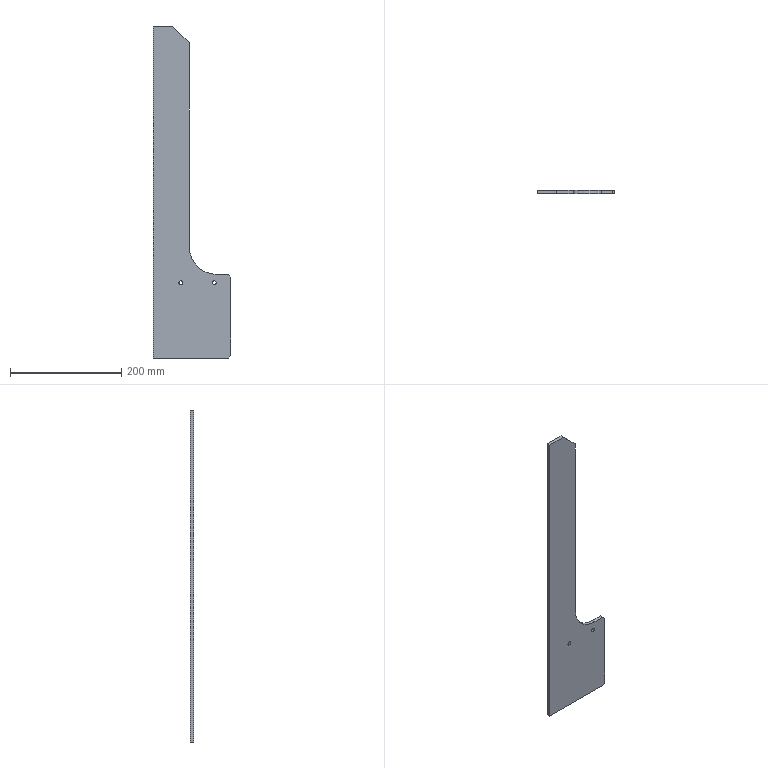Component | SolidWorks | THK-A1012BottomRibPlateRight-3 | 1 solid | 16 faces | box 140 x 6 x 596 mm | volume 299873 mm3 | plane 11 | cylinder 5 | commonest cylinder face diameters 6.8 x4 100 x1 | material Q235A
build123d program:
from build123d import *

# Parameters (mm, degrees)
BOSS_EXTRUDE1_DEPTH = 3
M8_TAPPED_HOLE1_D   = 6.8
CHAMFER2_SIZE       = 5
CHAMFER1_SIZE       = 30


with BuildPart() as part:
    # Sketch1 → Boss-Extrude1 (new, symmetric)
    with BuildSketch(Plane(origin=(0, 0, 0), x_dir=(1, 0, 0), z_dir=(0, 1, 0))):
        with BuildLine():
            Line((0, 0), (0, -596))
            Line((0, -596), (-65, -596))
            Line((-65, -596), (-65, -200))
            ThreePointArc((-65, -200), (-79.645, -164.645), (-115, -150))
            Line((-115, -150), (-140, -150))
            Line((-140, -150), (-140, 0))
            Line((-140, 0), (0, 0))
        make_face()
    extrude(amount=BOSS_EXTRUDE1_DEPTH, both=True)

    # M8 Tapped Hole1 (through all)
    with Locations(Plane(origin=(0, 3, 0), x_dir=(1, 0, 0), z_dir=(0, 1, 0))):
        with Locations((-110, -135), (-50, -135)):
            Hole(M8_TAPPED_HOLE1_D / 2)

    # Chamfer2
    chamfer2_edges = [part.edges().sort_by_distance(p)[0] for p in [
        (-140, 0, 150),
        (-140, 0, 0),
    ]]
    chamfer(chamfer2_edges, length=CHAMFER2_SIZE)

    # Chamfer1
    chamfer1_edges = [part.edges().sort_by_distance(p)[0] for p in [
        (-65, 0, 596),
    ]]
    chamfer(chamfer1_edges, length=CHAMFER1_SIZE)


solid = part.part

# Placed as in the assembly
solid = solid.moved(Location((73, -158, -371), (0, 0, 180)))
STEP:
#1=CARTESIAN_POINT('',(7.205,-6.102,-9.425));
#2=VERTEX_POINT('',#1);
#3=CARTESIAN_POINT('',(7.205,-6.102,-9.157));
#4=VERTEX_POINT('',#3);
#5=CARTESIAN_POINT('',(7.205,-6.102,-9.291));
#6=DIRECTION('',(0.,-1.,0.));
#7=DIRECTION('',(0.,0.,1.));
#8=AXIS2_PLACEMENT_3D('',#5,#6,#7);
#9=CIRCLE('',#8,0.1339);
#10=EDGE_CURVE('',#2,#4,#9,.T.);
#11=ORIENTED_EDGE('',*,*,#10,.F.);
#12=CARTESIAN_POINT('',(7.205,-6.339,-9.425));
#13=VERTEX_POINT('',#12);
#14=CARTESIAN_POINT('',(7.205,-6.339,-9.425));
#15=DIRECTION('',(0.,-1.,0.));
#16=VECTOR('',#15,39.37);
#17=LINE('',#14,#16);
#18=EDGE_CURVE('',#2,#13,#17,.T.);
#19=ORIENTED_EDGE('',*,*,#18,.T.);
#20=CARTESIAN_POINT('',(7.205,-6.339,-9.157));
#21=VERTEX_POINT('',#20);
#22=CARTESIAN_POINT('',(7.205,-6.339,-9.291));
#23=DIRECTION('',(0.,-1.,0.));
#24=DIRECTION('',(0.,0.,1.));
#25=AXIS2_PLACEMENT_3D('',#22,#23,#24);
#26=CIRCLE('',#25,0.1339);
#27=EDGE_CURVE('',#13,#21,#26,.T.);
#28=ORIENTED_EDGE('',*,*,#27,.T.);
#29=CARTESIAN_POINT('',(7.205,-6.339,-9.157));
#30=DIRECTION('',(0.,-1.,0.));
#31=VECTOR('',#30,39.37);
#32=LINE('',#29,#31);
#33=EDGE_CURVE('',#4,#21,#32,.T.);
#34=ORIENTED_EDGE('',*,*,#33,.F.);
#35=EDGE_LOOP('',(#11,#19,#28,#34));
#36=FACE_OUTER_BOUND('',#35,.T.);
#37=CARTESIAN_POINT('',(7.205,-6.339,-9.291));
#38=DIRECTION('',(0.,-1.,0.));
#39=DIRECTION('',(0.,0.,1.));
#40=AXIS2_PLACEMENT_3D('',#37,#38,#39);
#41=CYLINDRICAL_SURFACE('',#40,0.1339);
#42=ADVANCED_FACE('',(#36),#41,.F.);
#43=CARTESIAN_POINT('',(4.843,-6.102,-9.425));
#44=VERTEX_POINT('',#43);
#45=CARTESIAN_POINT('',(4.843,-6.102,-9.157));
#46=VERTEX_POINT('',#45);
#47=CARTESIAN_POINT('',(4.843,-6.102,-9.291));
#48=DIRECTION('',(0.,-1.,0.));
#49=DIRECTION('',(0.,0.,1.));
#50=AXIS2_PLACEMENT_3D('',#47,#48,#49);
#51=CIRCLE('',#50,0.1339);
#52=EDGE_CURVE('',#44,#46,#51,.T.);
#53=ORIENTED_EDGE('',*,*,#52,.F.);
#54=CARTESIAN_POINT('',(4.843,-6.339,-9.425));
#55=VERTEX_POINT('',#54);
#56=CARTESIAN_POINT('',(4.843,-6.339,-9.425));
#57=DIRECTION('',(0.,-1.,0.));
#58=VECTOR('',#57,39.37);
#59=LINE('',#56,#58);
#60=EDGE_CURVE('',#44,#55,#59,.T.);
#61=ORIENTED_EDGE('',*,*,#60,.T.);
#62=CARTESIAN_POINT('',(4.843,-6.339,-9.157));
#63=VERTEX_POINT('',#62);
#64=CARTESIAN_POINT('',(4.843,-6.339,-9.291));
#65=DIRECTION('',(0.,-1.,0.));
#66=DIRECTION('',(0.,0.,1.));
#67=AXIS2_PLACEMENT_3D('',#64,#65,#66);
#68=CIRCLE('',#67,0.1339);
#69=EDGE_CURVE('',#55,#63,#68,.T.);
#70=ORIENTED_EDGE('',*,*,#69,.T.);
#71=CARTESIAN_POINT('',(4.843,-6.339,-9.157));
#72=DIRECTION('',(0.,-1.,0.));
#73=VECTOR('',#72,39.37);
#74=LINE('',#71,#73);
#75=EDGE_CURVE('',#46,#63,#74,.T.);
#76=ORIENTED_EDGE('',*,*,#75,.F.);
#77=EDGE_LOOP('',(#53,#61,#70,#76));
#78=FACE_OUTER_BOUND('',#77,.T.);
#79=CARTESIAN_POINT('',(4.843,-6.339,-9.291));
#80=DIRECTION('',(0.,-1.,0.));
#81=DIRECTION('',(0.,0.,1.));
#82=AXIS2_PLACEMENT_3D('',#79,#80,#81);
#83=CYLINDRICAL_SURFACE('',#82,0.1339);
#84=ADVANCED_FACE('',(#78),#83,.F.);
#85=CARTESIAN_POINT('',(2.874,-6.102,-14.606));
#86=VERTEX_POINT('',#85);
#87=CARTESIAN_POINT('',(8.189,-6.102,-14.606));
#88=VERTEX_POINT('',#87);
#89=CARTESIAN_POINT('',(2.874,-6.102,-14.606));
#90=DIRECTION('',(1.,0.,-0.));
#91=VECTOR('',#90,39.37);
#92=LINE('',#89,#91);
#93=EDGE_CURVE('',#86,#88,#92,.T.);
#94=ORIENTED_EDGE('',*,*,#93,.T.);
#95=CARTESIAN_POINT('',(8.189,-6.339,-14.606));
#96=VERTEX_POINT('',#95);
#97=CARTESIAN_POINT('',(8.189,-6.339,-14.606));
#98=DIRECTION('',(0.,-1.,0.));
#99=VECTOR('',#98,39.37);
#100=LINE('',#97,#99);
#101=EDGE_CURVE('',#88,#96,#100,.T.);
#102=ORIENTED_EDGE('',*,*,#101,.T.);
#103=CARTESIAN_POINT('',(2.874,-6.339,-14.606));
#104=VERTEX_POINT('',#103);
#105=CARTESIAN_POINT('',(2.874,-6.339,-14.606));
#106=DIRECTION('',(1.,0.,-0.));
#107=VECTOR('',#106,39.37);
#108=LINE('',#105,#107);
#109=EDGE_CURVE('',#104,#96,#108,.T.);
#110=ORIENTED_EDGE('',*,*,#109,.F.);
#111=CARTESIAN_POINT('',(2.874,-6.339,-14.606));
#112=DIRECTION('',(-0.,1.,-0.));
#113=VECTOR('',#112,39.37);
#114=LINE('',#111,#113);
#115=EDGE_CURVE('',#104,#86,#114,.T.);
#116=ORIENTED_EDGE('',*,*,#115,.T.);
#117=EDGE_LOOP('',(#94,#102,#110,#116));
#118=FACE_OUTER_BOUND('',#117,.T.);
#119=CARTESIAN_POINT('',(2.874,-6.339,-14.606));
#120=DIRECTION('',(0.,0.,1.));
#121=DIRECTION('',(-1.,-0.,0.));
#122=AXIS2_PLACEMENT_3D('',#119,#120,#121);
#123=PLANE('',#122);
#124=ADVANCED_FACE('',(#118),#123,.F.);
#125=CARTESIAN_POINT('',(8.386,-6.102,-14.409));
#126=VERTEX_POINT('',#125);
#127=CARTESIAN_POINT('',(8.386,-6.102,-8.898));
#128=VERTEX_POINT('',#127);
#129=CARTESIAN_POINT('',(8.386,-6.102,-14.606));
#130=DIRECTION('',(0.,0.,1.));
#131=VECTOR('',#130,39.37);
#132=LINE('',#129,#131);
#133=EDGE_CURVE('',#126,#128,#132,.T.);
#134=ORIENTED_EDGE('',*,*,#133,.T.);
#135=CARTESIAN_POINT('',(8.386,-6.339,-8.898));
#136=VERTEX_POINT('',#135);
#137=CARTESIAN_POINT('',(8.386,-6.339,-8.898));
#138=DIRECTION('',(0.,-1.,0.));
#139=VECTOR('',#138,39.37);
#140=LINE('',#137,#139);
#141=EDGE_CURVE('',#128,#136,#140,.T.);
#142=ORIENTED_EDGE('',*,*,#141,.T.);
#143=CARTESIAN_POINT('',(8.386,-6.339,-14.409));
#144=VERTEX_POINT('',#143);
#145=CARTESIAN_POINT('',(8.386,-6.339,-14.606));
#146=DIRECTION('',(0.,0.,1.));
#147=VECTOR('',#146,39.37);
#148=LINE('',#145,#147);
#149=EDGE_CURVE('',#144,#136,#148,.T.);
#150=ORIENTED_EDGE('',*,*,#149,.F.);
#151=CARTESIAN_POINT('',(8.386,-6.339,-14.409));
#152=DIRECTION('',(-0.,1.,-0.));
#153=VECTOR('',#152,39.37);
#154=LINE('',#151,#153);
#155=EDGE_CURVE('',#144,#126,#154,.T.);
#156=ORIENTED_EDGE('',*,*,#155,.T.);
#157=EDGE_LOOP('',(#134,#142,#150,#156));
#158=FACE_OUTER_BOUND('',#157,.T.);
#159=CARTESIAN_POINT('',(8.386,-6.339,-14.606));
#160=DIRECTION('',(-1.,-0.,0.));
#161=DIRECTION('',(-0.,-0.,-1.));
#162=AXIS2_PLACEMENT_3D('',#159,#160,#161);
#163=PLANE('',#162);
#164=ADVANCED_FACE('',(#158),#163,.F.);
#165=CARTESIAN_POINT('',(8.189,-6.339,-8.701));
#166=VERTEX_POINT('',#165);
#167=CARTESIAN_POINT('',(7.402,-6.339,-8.701));
#168=VERTEX_POINT('',#167);
#169=CARTESIAN_POINT('',(8.386,-6.339,-8.701));
#170=DIRECTION('',(-1.,-0.,0.));
#171=VECTOR('',#170,39.37);
#172=LINE('',#169,#171);
#173=EDGE_CURVE('',#166,#168,#172,.T.);
#174=ORIENTED_EDGE('',*,*,#173,.F.);
#175=CARTESIAN_POINT('',(8.189,-6.102,-8.701));
#176=VERTEX_POINT('',#175);
#177=CARTESIAN_POINT('',(8.189,-6.339,-8.701));
#178=DIRECTION('',(-0.,1.,-0.));
#179=VECTOR('',#178,39.37);
#180=LINE('',#177,#179);
#181=EDGE_CURVE('',#166,#176,#180,.T.);
#182=ORIENTED_EDGE('',*,*,#181,.T.);
#183=CARTESIAN_POINT('',(7.402,-6.102,-8.701));
#184=VERTEX_POINT('',#183);
#185=CARTESIAN_POINT('',(8.386,-6.102,-8.701));
#186=DIRECTION('',(-1.,-0.,0.));
#187=VECTOR('',#186,39.37);
#188=LINE('',#185,#187);
#189=EDGE_CURVE('',#176,#184,#188,.T.);
#190=ORIENTED_EDGE('',*,*,#189,.T.);
#191=CARTESIAN_POINT('',(7.402,-6.339,-8.701));
#192=DIRECTION('',(-0.,1.,-0.));
#193=VECTOR('',#192,39.37);
#194=LINE('',#191,#193);
#195=EDGE_CURVE('',#168,#184,#194,.T.);
#196=ORIENTED_EDGE('',*,*,#195,.F.);
#197=EDGE_LOOP('',(#174,#182,#190,#196));
#198=FACE_OUTER_BOUND('',#197,.T.);
#199=CARTESIAN_POINT('',(8.386,-6.339,-8.701));
#200=DIRECTION('',(-0.,-0.,-1.));
#201=DIRECTION('',(1.,0.,-0.));
#202=AXIS2_PLACEMENT_3D('',#199,#200,#201);
#203=PLANE('',#202);
#204=ADVANCED_FACE('',(#198),#203,.F.);
#205=CARTESIAN_POINT('',(5.433,-6.102,-6.732));
#206=VERTEX_POINT('',#205);
#207=CARTESIAN_POINT('',(7.402,-6.102,-6.732));
#208=DIRECTION('',(-0.,1.,-0.));
#209=DIRECTION('',(0.,0.,1.));
#210=AXIS2_PLACEMENT_3D('',#207,#208,#209);
#211=CIRCLE('',#210,1.969);
#212=EDGE_CURVE('',#184,#206,#211,.T.);
#213=ORIENTED_EDGE('',*,*,#212,.T.);
#214=CARTESIAN_POINT('',(5.433,-6.339,-6.732));
#215=VERTEX_POINT('',#214);
#216=CARTESIAN_POINT('',(5.433,-6.339,-6.732));
#217=DIRECTION('',(-0.,1.,-0.));
#218=VECTOR('',#217,39.37);
#219=LINE('',#216,#218);
#220=EDGE_CURVE('',#215,#206,#219,.T.);
#221=ORIENTED_EDGE('',*,*,#220,.F.);
#222=CARTESIAN_POINT('',(7.402,-6.339,-6.732));
#223=DIRECTION('',(-0.,1.,-0.));
#224=DIRECTION('',(0.,0.,1.));
#225=AXIS2_PLACEMENT_3D('',#222,#223,#224);
#226=CIRCLE('',#225,1.969);
#227=EDGE_CURVE('',#168,#215,#226,.T.);
#228=ORIENTED_EDGE('',*,*,#227,.F.);
#229=ORIENTED_EDGE('',*,*,#195,.T.);
#230=EDGE_LOOP('',(#213,#221,#228,#229));
#231=FACE_OUTER_BOUND('',#230,.T.);
#232=CARTESIAN_POINT('',(7.402,-6.339,-6.732));
#233=DIRECTION('',(-0.,1.,-0.));
#234=DIRECTION('',(0.,0.,-1.));
#235=AXIS2_PLACEMENT_3D('',#232,#233,#234);
#236=CYLINDRICAL_SURFACE('',#235,1.969);
#237=ADVANCED_FACE('',(#231),#236,.F.);
#238=CARTESIAN_POINT('',(5.433,-6.102,7.677));
#239=VERTEX_POINT('',#238);
#240=CARTESIAN_POINT('',(5.433,-6.102,-6.732));
#241=DIRECTION('',(0.,0.,1.));
#242=VECTOR('',#241,39.37);
#243=LINE('',#240,#242);
#244=EDGE_CURVE('',#206,#239,#243,.T.);
#245=ORIENTED_EDGE('',*,*,#244,.T.);
#246=CARTESIAN_POINT('',(5.433,-6.339,7.677));
#247=VERTEX_POINT('',#246);
#248=CARTESIAN_POINT('',(5.433,-6.339,7.677));
#249=DIRECTION('',(0.,-1.,0.));
#250=VECTOR('',#249,39.37);
#251=LINE('',#248,#250);
#252=EDGE_CURVE('',#239,#247,#251,.T.);
#253=ORIENTED_EDGE('',*,*,#252,.T.);
#254=CARTESIAN_POINT('',(5.433,-6.339,-6.732));
#255=DIRECTION('',(0.,0.,1.));
#256=VECTOR('',#255,39.37);
#257=LINE('',#254,#256);
#258=EDGE_CURVE('',#215,#247,#257,.T.);
#259=ORIENTED_EDGE('',*,*,#258,.F.);
#260=ORIENTED_EDGE('',*,*,#220,.T.);
#261=EDGE_LOOP('',(#245,#253,#259,#260));
#262=FACE_OUTER_BOUND('',#261,.T.);
#263=CARTESIAN_POINT('',(5.433,-6.339,-6.732));
#264=DIRECTION('',(-1.,-0.,0.));
#265=DIRECTION('',(-0.,-0.,-1.));
#266=AXIS2_PLACEMENT_3D('',#263,#264,#265);
#267=PLANE('',#266);
#268=ADVANCED_FACE('',(#262),#267,.F.);
#269=CARTESIAN_POINT('',(4.252,-6.339,8.858));
#270=VERTEX_POINT('',#269);
#271=CARTESIAN_POINT('',(2.874,-6.339,8.858));
#272=VERTEX_POINT('',#271);
#273=CARTESIAN_POINT('',(5.433,-6.339,8.858));
#274=DIRECTION('',(-1.,-0.,0.));
#275=VECTOR('',#274,39.37);
#276=LINE('',#273,#275);
#277=EDGE_CURVE('',#270,#272,#276,.T.);
#278=ORIENTED_EDGE('',*,*,#277,.F.);
#279=CARTESIAN_POINT('',(4.252,-6.102,8.858));
#280=VERTEX_POINT('',#279);
#281=CARTESIAN_POINT('',(4.252,-6.339,8.858));
#282=DIRECTION('',(-0.,1.,-0.));
#283=VECTOR('',#282,39.37);
#284=LINE('',#281,#283);
#285=EDGE_CURVE('',#270,#280,#284,.T.);
#286=ORIENTED_EDGE('',*,*,#285,.T.);
#287=CARTESIAN_POINT('',(2.874,-6.102,8.858));
#288=VERTEX_POINT('',#287);
#289=CARTESIAN_POINT('',(5.433,-6.102,8.858));
#290=DIRECTION('',(-1.,-0.,0.));
#291=VECTOR('',#290,39.37);
#292=LINE('',#289,#291);
#293=EDGE_CURVE('',#280,#288,#292,.T.);
#294=ORIENTED_EDGE('',*,*,#293,.T.);
#295=CARTESIAN_POINT('',(2.874,-6.339,8.858));
#296=DIRECTION('',(-0.,1.,-0.));
#297=VECTOR('',#296,39.37);
#298=LINE('',#295,#297);
#299=EDGE_CURVE('',#272,#288,#298,.T.);
#300=ORIENTED_EDGE('',*,*,#299,.F.);
#301=EDGE_LOOP('',(#278,#286,#294,#300));
#302=FACE_OUTER_BOUND('',#301,.T.);
#303=CARTESIAN_POINT('',(5.433,-6.339,8.858));
#304=DIRECTION('',(-0.,-0.,-1.));
#305=DIRECTION('',(1.,0.,-0.));
#306=AXIS2_PLACEMENT_3D('',#303,#304,#305);
#307=PLANE('',#306);
#308=ADVANCED_FACE('',(#302),#307,.F.);
#309=CARTESIAN_POINT('',(2.874,-6.102,-14.606));
#310=DIRECTION('',(-0.,-0.,-1.));
#311=VECTOR('',#310,39.37);
#312=LINE('',#309,#311);
#313=EDGE_CURVE('',#288,#86,#312,.T.);
#314=ORIENTED_EDGE('',*,*,#313,.T.);
#315=ORIENTED_EDGE('',*,*,#115,.F.);
#316=CARTESIAN_POINT('',(2.874,-6.339,-14.606));
#317=DIRECTION('',(-0.,-0.,-1.));
#318=VECTOR('',#317,39.37);
#319=LINE('',#316,#318);
#320=EDGE_CURVE('',#272,#104,#319,.T.);
#321=ORIENTED_EDGE('',*,*,#320,.F.);
#322=ORIENTED_EDGE('',*,*,#299,.T.);
#323=EDGE_LOOP('',(#314,#315,#321,#322));
#324=FACE_OUTER_BOUND('',#323,.T.);
#325=CARTESIAN_POINT('',(2.874,-6.339,-14.606));
#326=DIRECTION('',(1.,0.,-0.));
#327=DIRECTION('',(0.,0.,1.));
#328=AXIS2_PLACEMENT_3D('',#325,#326,#327);
#329=PLANE('',#328);
#330=ADVANCED_FACE('',(#324),#329,.F.);
#331=CARTESIAN_POINT('',(7.205,-6.339,-9.291));
#332=DIRECTION('',(0.,-1.,0.));
#333=DIRECTION('',(0.,0.,1.));
#334=AXIS2_PLACEMENT_3D('',#331,#332,#333);
#335=CIRCLE('',#334,0.1339);
#336=EDGE_CURVE('',#21,#13,#335,.T.);
#337=ORIENTED_EDGE('',*,*,#336,.F.);
#338=ORIENTED_EDGE('',*,*,#27,.F.);
#339=EDGE_LOOP('',(#337,#338));
#340=FACE_BOUND('',#339,.T.);
#341=CARTESIAN_POINT('',(4.843,-6.339,-9.291));
#342=DIRECTION('',(0.,-1.,0.));
#343=DIRECTION('',(0.,0.,1.));
#344=AXIS2_PLACEMENT_3D('',#341,#342,#343);
#345=CIRCLE('',#344,0.1339);
#346=EDGE_CURVE('',#63,#55,#345,.T.);
#347=ORIENTED_EDGE('',*,*,#346,.F.);
#348=ORIENTED_EDGE('',*,*,#69,.F.);
#349=EDGE_LOOP('',(#347,#348));
#350=FACE_BOUND('',#349,.T.);
#351=ORIENTED_EDGE('',*,*,#258,.T.);
#352=CARTESIAN_POINT('',(13.622,-6.339,-0.5118));
#353=DIRECTION('',(-0.7071,-0.,0.7071));
#354=VECTOR('',#353,39.37);
#355=LINE('',#352,#354);
#356=EDGE_CURVE('',#247,#270,#355,.T.);
#357=ORIENTED_EDGE('',*,*,#356,.T.);
#358=ORIENTED_EDGE('',*,*,#277,.T.);
#359=ORIENTED_EDGE('',*,*,#320,.T.);
#360=ORIENTED_EDGE('',*,*,#109,.T.);
#361=CARTESIAN_POINT('',(11.732,-6.339,-11.063));
#362=DIRECTION('',(0.7071,0.,0.7071));
#363=VECTOR('',#362,39.37);
#364=LINE('',#361,#363);
#365=EDGE_CURVE('',#96,#144,#364,.T.);
#366=ORIENTED_EDGE('',*,*,#365,.T.);
#367=ORIENTED_EDGE('',*,*,#149,.T.);
#368=CARTESIAN_POINT('',(6.811,-6.339,-7.323));
#369=DIRECTION('',(-0.7071,-0.,0.7071));
#370=VECTOR('',#369,39.37);
#371=LINE('',#368,#370);
#372=EDGE_CURVE('',#136,#166,#371,.T.);
#373=ORIENTED_EDGE('',*,*,#372,.T.);
#374=ORIENTED_EDGE('',*,*,#173,.T.);
#375=ORIENTED_EDGE('',*,*,#227,.T.);
#376=EDGE_LOOP('',(#351,#357,#358,#359,#360,#366,#367,#373,#374,#375));
#377=FACE_OUTER_BOUND('',#376,.T.);
#378=CARTESIAN_POINT('',(7.402,-6.339,-6.732));
#379=DIRECTION('',(0.,-1.,0.));
#380=DIRECTION('',(0.,0.,1.));
#381=AXIS2_PLACEMENT_3D('',#378,#379,#380);
#382=PLANE('',#381);
#383=ADVANCED_FACE('',(#340,#350,#377),#382,.T.);
#384=CARTESIAN_POINT('',(7.205,-6.102,-9.291));
#385=DIRECTION('',(0.,-1.,0.));
#386=DIRECTION('',(0.,0.,1.));
#387=AXIS2_PLACEMENT_3D('',#384,#385,#386);
#388=CIRCLE('',#387,0.1339);
#389=EDGE_CURVE('',#4,#2,#388,.T.);
#390=ORIENTED_EDGE('',*,*,#389,.T.);
#391=ORIENTED_EDGE('',*,*,#10,.T.);
#392=EDGE_LOOP('',(#390,#391));
#393=FACE_BOUND('',#392,.T.);
#394=CARTESIAN_POINT('',(4.843,-6.102,-9.291));
#395=DIRECTION('',(0.,-1.,0.));
#396=DIRECTION('',(0.,0.,1.));
#397=AXIS2_PLACEMENT_3D('',#394,#395,#396);
#398=CIRCLE('',#397,0.1339);
#399=EDGE_CURVE('',#46,#44,#398,.T.);
#400=ORIENTED_EDGE('',*,*,#399,.T.);
#401=ORIENTED_EDGE('',*,*,#52,.T.);
#402=EDGE_LOOP('',(#400,#401));
#403=FACE_BOUND('',#402,.T.);
#404=ORIENTED_EDGE('',*,*,#293,.F.);
#405=CARTESIAN_POINT('',(4.252,-6.102,8.858));
#406=DIRECTION('',(0.7071,0.,-0.7071));
#407=VECTOR('',#406,39.37);
#408=LINE('',#405,#407);
#409=EDGE_CURVE('',#280,#239,#408,.T.);
#410=ORIENTED_EDGE('',*,*,#409,.T.);
#411=ORIENTED_EDGE('',*,*,#244,.F.);
#412=ORIENTED_EDGE('',*,*,#212,.F.);
#413=ORIENTED_EDGE('',*,*,#189,.F.);
#414=CARTESIAN_POINT('',(8.189,-6.102,-8.701));
#415=DIRECTION('',(0.7071,0.,-0.7071));
#416=VECTOR('',#415,39.37);
#417=LINE('',#414,#416);
#418=EDGE_CURVE('',#176,#128,#417,.T.);
#419=ORIENTED_EDGE('',*,*,#418,.T.);
#420=ORIENTED_EDGE('',*,*,#133,.F.);
#421=CARTESIAN_POINT('',(8.386,-6.102,-14.409));
#422=DIRECTION('',(-0.7071,-0.,-0.7071));
#423=VECTOR('',#422,39.37);
#424=LINE('',#421,#423);
#425=EDGE_CURVE('',#126,#88,#424,.T.);
#426=ORIENTED_EDGE('',*,*,#425,.T.);
#427=ORIENTED_EDGE('',*,*,#93,.F.);
#428=ORIENTED_EDGE('',*,*,#313,.F.);
#429=EDGE_LOOP('',(#404,#410,#411,#412,#413,#419,#420,#426,#427,#428));
#430=FACE_OUTER_BOUND('',#429,.T.);
#431=CARTESIAN_POINT('',(7.402,-6.102,-6.732));
#432=DIRECTION('',(0.,-1.,0.));
#433=DIRECTION('',(0.,0.,1.));
#434=AXIS2_PLACEMENT_3D('',#431,#432,#433);
#435=PLANE('',#434);
#436=ADVANCED_FACE('',(#393,#403,#430),#435,.F.);
#437=ORIENTED_EDGE('',*,*,#60,.F.);
#438=ORIENTED_EDGE('',*,*,#399,.F.);
#439=ORIENTED_EDGE('',*,*,#75,.T.);
#440=ORIENTED_EDGE('',*,*,#346,.T.);
#441=EDGE_LOOP('',(#437,#438,#439,#440));
#442=FACE_OUTER_BOUND('',#441,.T.);
#443=CARTESIAN_POINT('',(4.843,-6.339,-9.291));
#444=DIRECTION('',(0.,-1.,0.));
#445=DIRECTION('',(0.,0.,1.));
#446=AXIS2_PLACEMENT_3D('',#443,#444,#445);
#447=CYLINDRICAL_SURFACE('',#446,0.1339);
#448=ADVANCED_FACE('',(#442),#447,.F.);
#449=ORIENTED_EDGE('',*,*,#18,.F.);
#450=ORIENTED_EDGE('',*,*,#389,.F.);
#451=ORIENTED_EDGE('',*,*,#33,.T.);
#452=ORIENTED_EDGE('',*,*,#336,.T.);
#453=EDGE_LOOP('',(#449,#450,#451,#452));
#454=FACE_OUTER_BOUND('',#453,.T.);
#455=CARTESIAN_POINT('',(7.205,-6.339,-9.291));
#456=DIRECTION('',(0.,-1.,0.));
#457=DIRECTION('',(0.,0.,1.));
#458=AXIS2_PLACEMENT_3D('',#455,#456,#457);
#459=CYLINDRICAL_SURFACE('',#458,0.1339);
#460=ADVANCED_FACE('',(#454),#459,.F.);
#461=ORIENTED_EDGE('',*,*,#372,.F.);
#462=ORIENTED_EDGE('',*,*,#141,.F.);
#463=ORIENTED_EDGE('',*,*,#418,.F.);
#464=ORIENTED_EDGE('',*,*,#181,.F.);
#465=EDGE_LOOP('',(#461,#462,#463,#464));
#466=FACE_OUTER_BOUND('',#465,.T.);
#467=CARTESIAN_POINT('',(8.189,-6.339,-8.701));
#468=DIRECTION('',(-0.7071,-0.,-0.7071));
#469=DIRECTION('',(-0.,1.,-0.));
#470=AXIS2_PLACEMENT_3D('',#467,#468,#469);
#471=PLANE('',#470);
#472=ADVANCED_FACE('',(#466),#471,.F.);
#473=ORIENTED_EDGE('',*,*,#365,.F.);
#474=ORIENTED_EDGE('',*,*,#101,.F.);
#475=ORIENTED_EDGE('',*,*,#425,.F.);
#476=ORIENTED_EDGE('',*,*,#155,.F.);
#477=EDGE_LOOP('',(#473,#474,#475,#476));
#478=FACE_OUTER_BOUND('',#477,.T.);
#479=CARTESIAN_POINT('',(8.386,-6.339,-14.409));
#480=DIRECTION('',(-0.7071,-0.,0.7071));
#481=DIRECTION('',(-0.,1.,-0.));
#482=AXIS2_PLACEMENT_3D('',#479,#480,#481);
#483=PLANE('',#482);
#484=ADVANCED_FACE('',(#478),#483,.F.);
#485=ORIENTED_EDGE('',*,*,#356,.F.);
#486=ORIENTED_EDGE('',*,*,#252,.F.);
#487=ORIENTED_EDGE('',*,*,#409,.F.);
#488=ORIENTED_EDGE('',*,*,#285,.F.);
#489=EDGE_LOOP('',(#485,#486,#487,#488));
#490=FACE_OUTER_BOUND('',#489,.T.);
#491=CARTESIAN_POINT('',(4.252,-6.339,8.858));
#492=DIRECTION('',(-0.7071,-0.,-0.7071));
#493=DIRECTION('',(-0.,1.,-0.));
#494=AXIS2_PLACEMENT_3D('',#491,#492,#493);
#495=PLANE('',#494);
#496=ADVANCED_FACE('',(#490),#495,.F.);
#497=CLOSED_SHELL('',(#42,#84,#124,#164,#204,#237,#268,#308,#330,#383,#436,#448,#460,#472,#484,#496));
#498=MANIFOLD_SOLID_BREP('',#497);
#499=CARTESIAN_POINT('',(0.,0.,0.));
#500=DIRECTION('',(0.,0.,1.));
#501=DIRECTION('',(1.,0.,0.));
#502=AXIS2_PLACEMENT_3D('',#499,#500,#501);
#503=(LENGTH_UNIT()NAMED_UNIT(*)SI_UNIT($,.METRE.));
#504=LENGTH_MEASURE_WITH_UNIT(LENGTH_MEASURE(0.0254),#503);
#505=DIMENSIONAL_EXPONENTS(1.,0.,0.,0.,0.,0.,0.);
#506=(CONVERSION_BASED_UNIT('',#504)LENGTH_UNIT()NAMED_UNIT(#505));
#507=UNCERTAINTY_MEASURE_WITH_UNIT(LENGTH_MEASURE(0.00001),#506,'','');
#508=(NAMED_UNIT(*)PLANE_ANGLE_UNIT()SI_UNIT($,.RADIAN.));
#509=(NAMED_UNIT(*)SI_UNIT($,.STERADIAN.)SOLID_ANGLE_UNIT());
#510=(GEOMETRIC_REPRESENTATION_CONTEXT(3)GLOBAL_UNCERTAINTY_ASSIGNED_CONTEXT((#507))GLOBAL_UNIT_ASSIGNED_CONTEXT((#506,#508,#509))REPRESENTATION_CONTEXT('',''));
#511=ADVANCED_BREP_SHAPE_REPRESENTATION('',(#498,#502),#510);
#512=COLOUR_RGB('',0.7922,0.8196,0.9333);
#513=FILL_AREA_STYLE_COLOUR('',#512);
#514=FILL_AREA_STYLE('',(#513));
#515=SURFACE_STYLE_FILL_AREA(#514);
#516=SURFACE_SIDE_STYLE('',(#515));
#517=SURFACE_STYLE_USAGE(.BOTH.,#516);
#518=PRESENTATION_STYLE_ASSIGNMENT((#517));
#519=STYLED_ITEM('',(#518),#498);
#520=PRESENTATION_LAYER_ASSIGNMENT('','',(#519));
#521=(LENGTH_UNIT()NAMED_UNIT(*)SI_UNIT($,.METRE.));
#522=LENGTH_MEASURE_WITH_UNIT(LENGTH_MEASURE(0.0254),#521);
#523=DIMENSIONAL_EXPONENTS(1.,0.,0.,0.,0.,0.,0.);
#524=(CONVERSION_BASED_UNIT('',#522)LENGTH_UNIT()NAMED_UNIT(#523));
#525=UNCERTAINTY_MEASURE_WITH_UNIT(LENGTH_MEASURE(0.00001),#524,'','');
#526=(NAMED_UNIT(*)PLANE_ANGLE_UNIT()SI_UNIT($,.RADIAN.));
#527=(NAMED_UNIT(*)SI_UNIT($,.STERADIAN.)SOLID_ANGLE_UNIT());
#528=(GEOMETRIC_REPRESENTATION_CONTEXT(3)GLOBAL_UNCERTAINTY_ASSIGNED_CONTEXT((#525))GLOBAL_UNIT_ASSIGNED_CONTEXT((#524,#526,#527))REPRESENTATION_CONTEXT('',''));
#529=MECHANICAL_DESIGN_GEOMETRIC_PRESENTATION_REPRESENTATION('',(#519),#528);